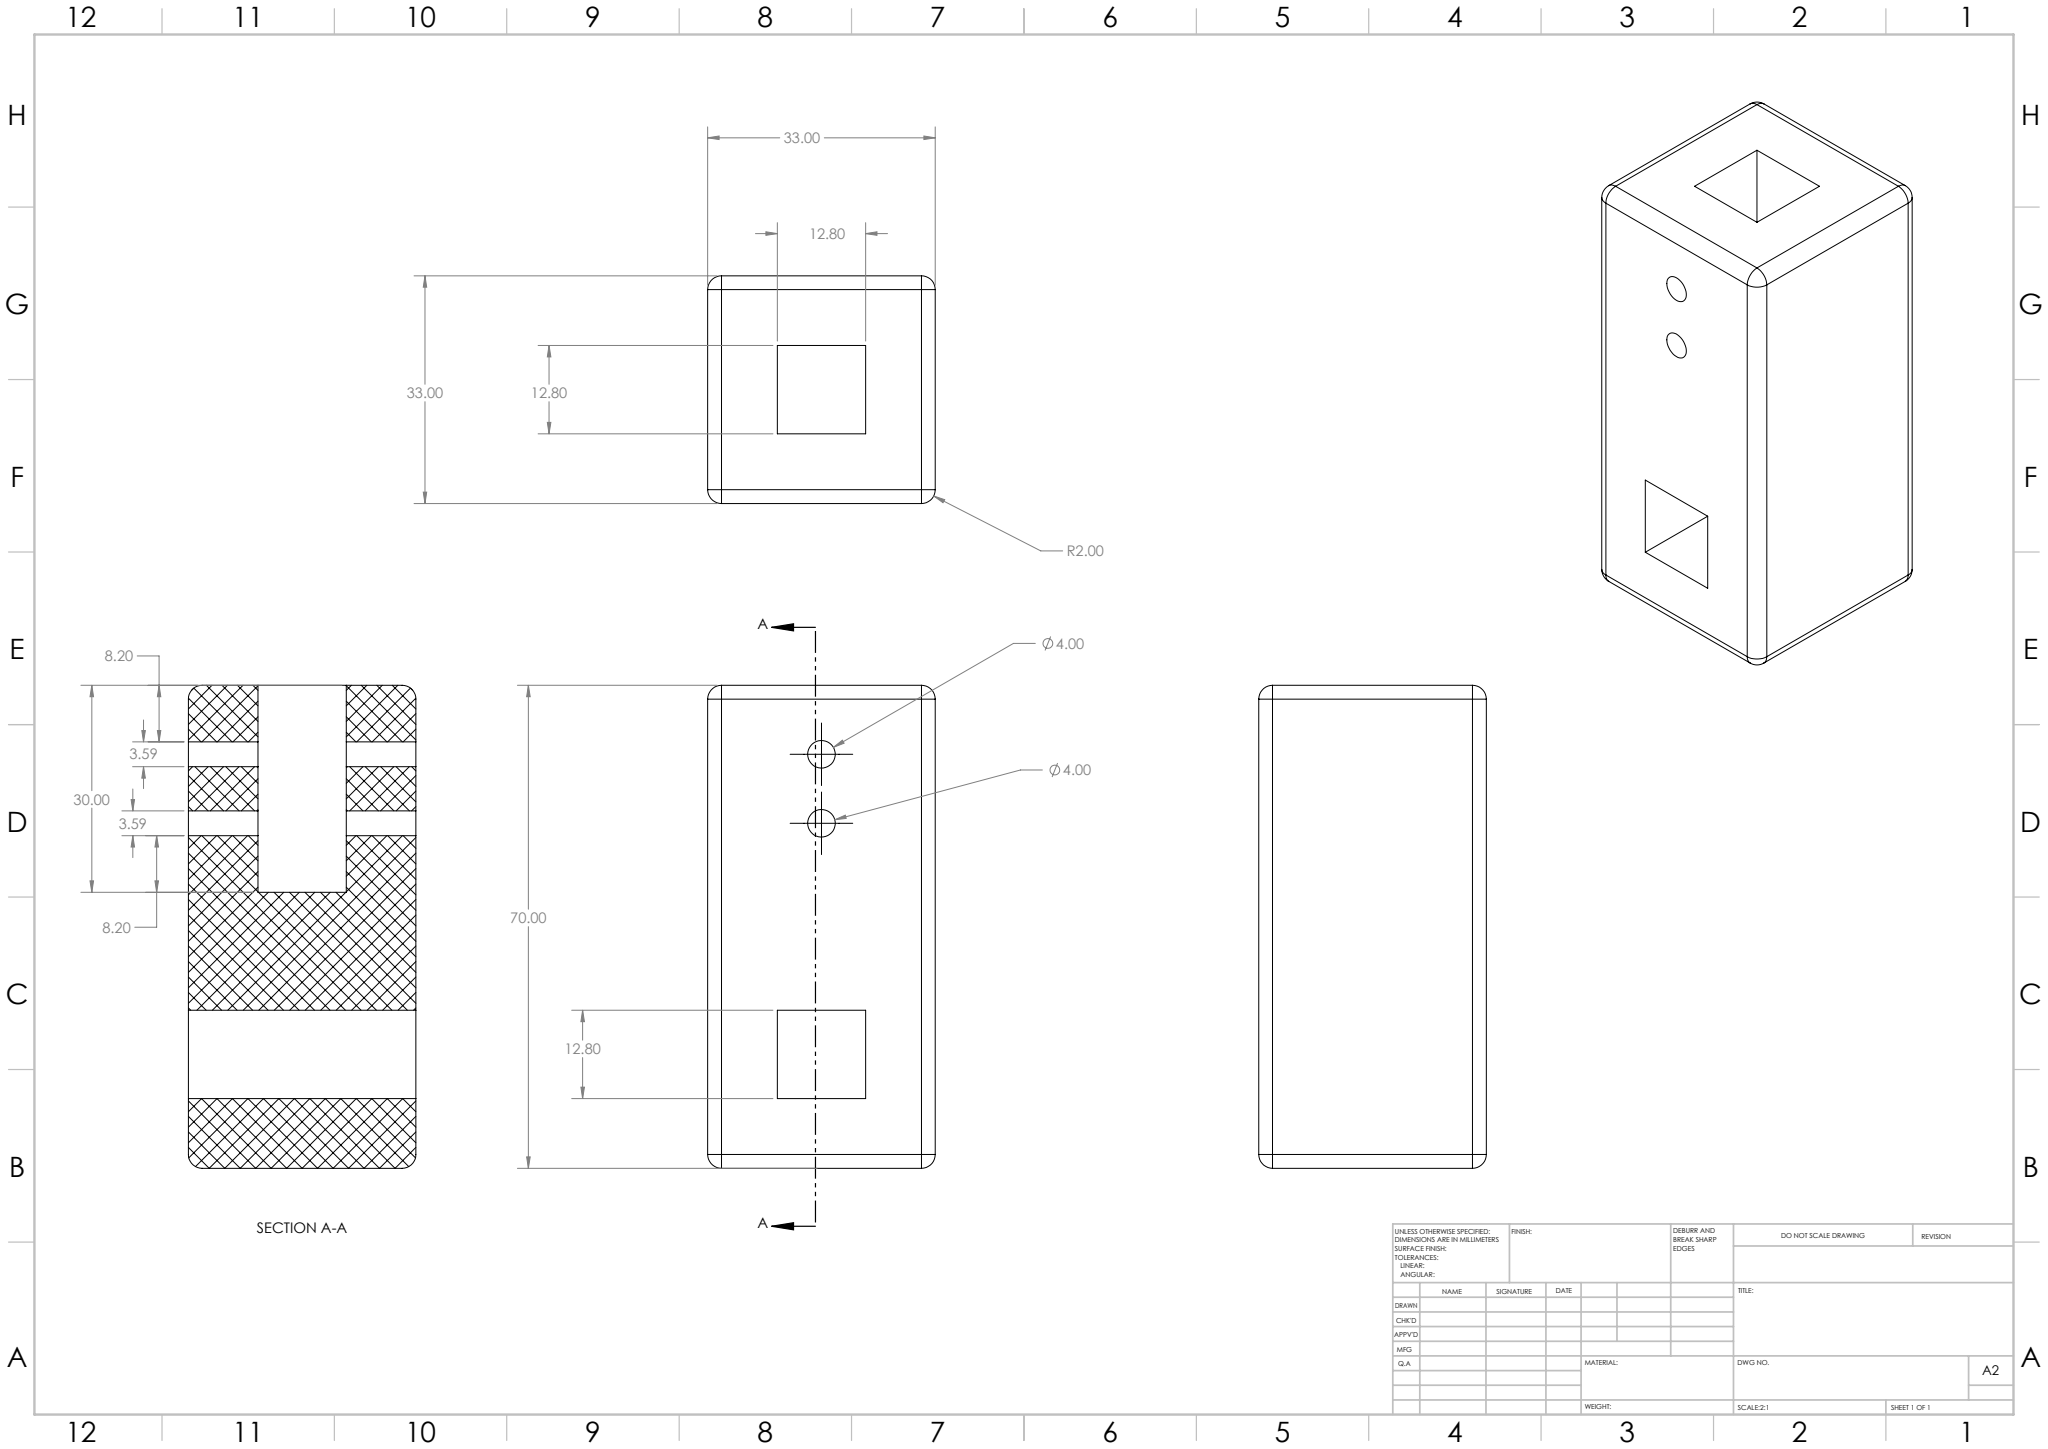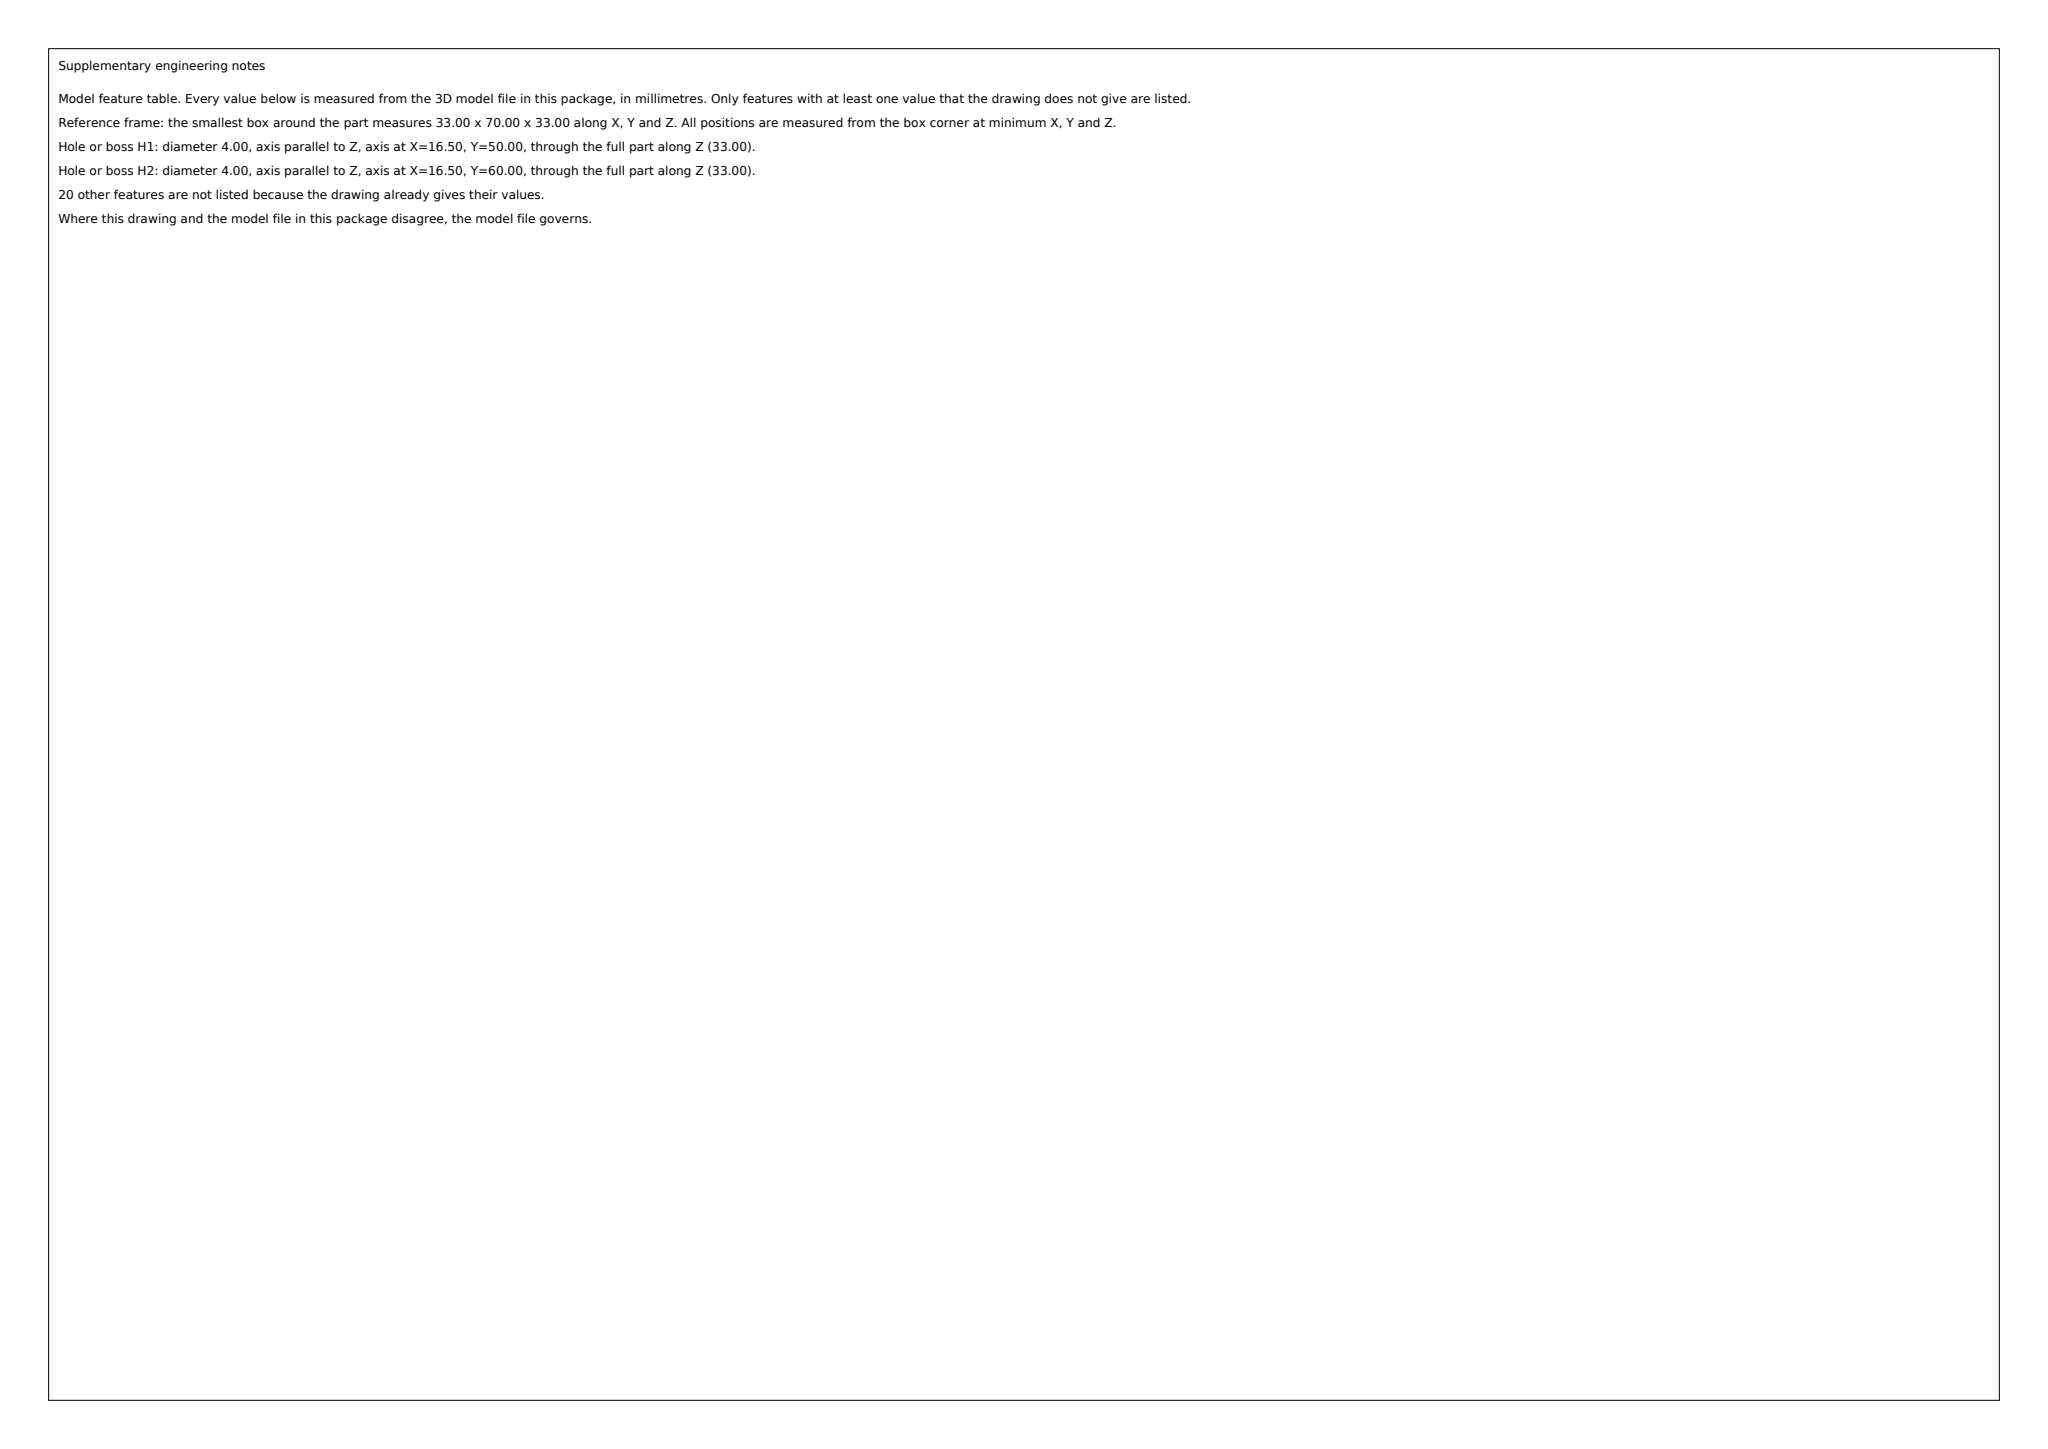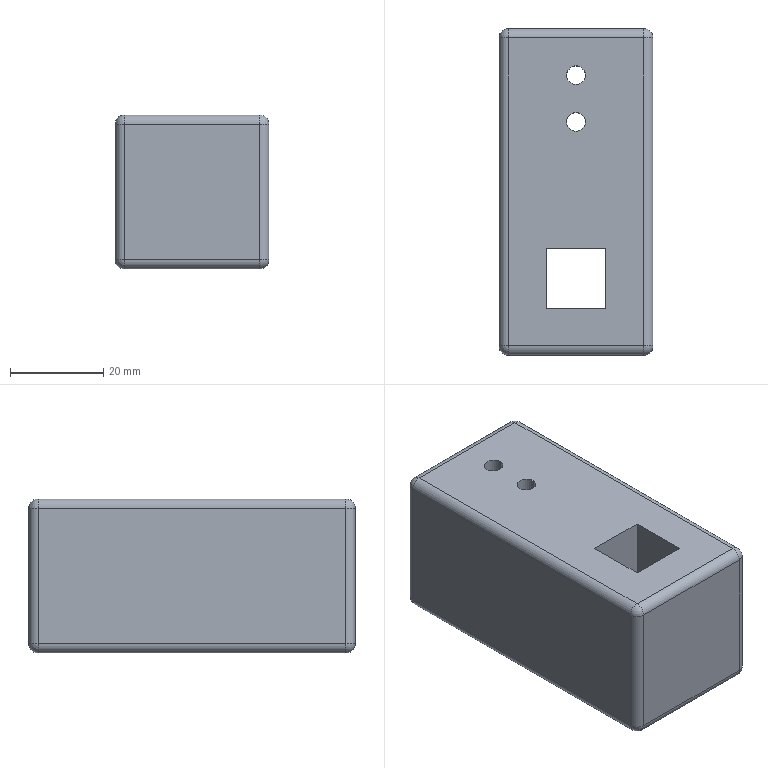Part | SolidWorks | mm | 1 solid | 43 faces | box 33 x 70 x 33 mm | volume 64944 mm3 | cylinder 20 | plane 15 | sphere 8 | commonest cylinder face diameters 4 x20
build123d program:
from build123d import *

# Parameters (mm, degrees)
SKETCH1_W           = 33
SKETCH1_H           = 33
BOSS_EXTRUDE1_DEPTH = 70
SKETCH2_W           = 12.8
SKETCH2_H           = 12.8
CUT_EXTRUDE1_DEPTH  = 80.128
SKETCH3_W           = 12.8
SKETCH3_H           = 12.8
CUT_EXTRUDE2_DEPTH  = 30
SKETCH4_R           = 2
CUT_EXTRUDE3_DEPTH  = 80.128
FILLET1_R           = 2


with BuildPart() as part:
    # Sketch1 → Boss-Extrude1 (new body)
    with BuildSketch(Plane(origin=(0, 0, 0), x_dir=(1, 0, 0), z_dir=(0, 1, 0))):
        Rectangle(SKETCH1_W, SKETCH1_H)
    extrude(amount=BOSS_EXTRUDE1_DEPTH)

    # Sketch2 → Cut-Extrude1 (cut, through all)
    with BuildSketch(Plane.XY.offset(16.5)):
        with Locations((0, 16.5)):
            Rectangle(SKETCH2_W, SKETCH2_H)
    extrude(amount=-CUT_EXTRUDE1_DEPTH, mode=Mode.SUBTRACT)

    # Sketch3 → Cut-Extrude2 (cut)
    with BuildSketch(Plane(origin=(0, 70, 0), x_dir=(1, 0, 0), z_dir=(0, 1, 0))):
        Rectangle(SKETCH3_W, SKETCH3_H)
    extrude(amount=-CUT_EXTRUDE2_DEPTH, mode=Mode.SUBTRACT)

    # Sketch4 → Cut-Extrude3 (cut, through all)
    with BuildSketch(Plane(origin=(0, 0, -16.5), x_dir=(-1, 0, 0), z_dir=(0, 0, -1))):
        with Locations((0, 60)):
            Circle(SKETCH4_R)
        with Locations((0, 50)):
            Circle(SKETCH4_R)
    extrude(amount=-CUT_EXTRUDE3_DEPTH, mode=Mode.SUBTRACT)

    # Fillet1
    fillet1_edges = [part.edges().sort_by_distance(p)[0] for p in [
        (-16.5, 70, 0),
        (0, 70, 16.5),
        (16.5, 70, 0),
        (0, 0, 16.5),
        (-16.5, 0, 0),
        (0, 0, -16.5),
        (16.5, 0, 0),
        (16.5, 35, 16.5),
        (-16.5, 35, 16.5),
        (-16.5, 35, -16.5),
        (16.5, 35, -16.5),
        (0, 70, -16.5),
    ]]
    fillet(fillet1_edges, radius=FILLET1_R)


solid = part.part